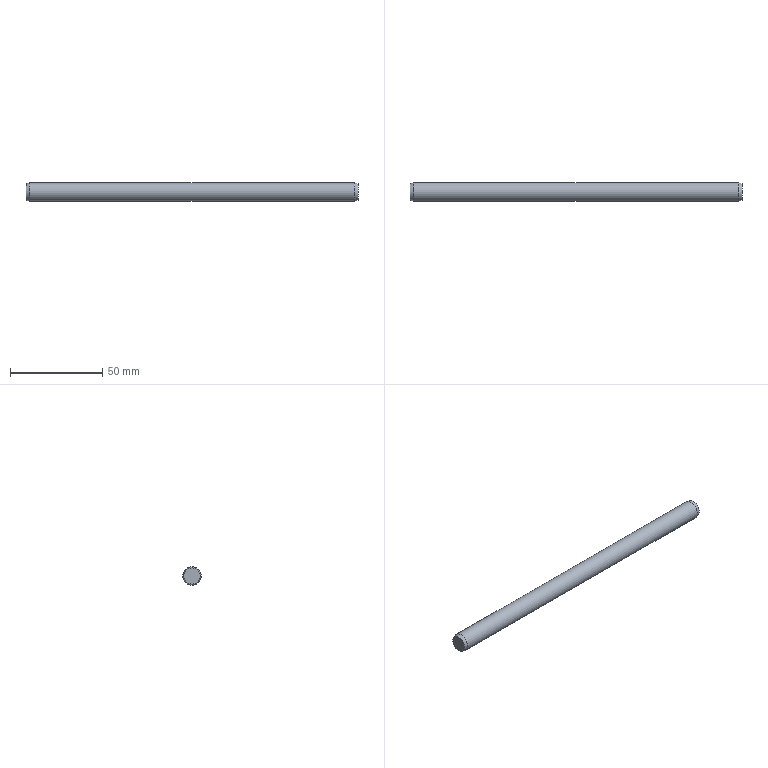Component | NX | HINGE | 1 solid | 5 faces | box 180 x 10 x 10 mm | volume 14105 mm3 | plane 2 | cone 2 | cylinder 1 | commonest cylinder face diameters 10 x1
STEP:
#1=CARTESIAN_POINT('',(0.,0.,0.));
#2=DIRECTION('',(0.,0.,1.));
#3=DIRECTION('',(1.,0.,0.));
#4=AXIS2_PLACEMENT_3D('',#1,#2,#3);
#5=CARTESIAN_POINT('',(-90.,140.,105.536));
#6=VERTEX_POINT('',#5);
#7=CARTESIAN_POINT('',(-90.,140.,110.));
#8=DIRECTION('',(-1.,0.,0.));
#9=DIRECTION('',(0.,0.,-1.));
#10=AXIS2_PLACEMENT_3D('',#7,#8,#9);
#11=CIRCLE('',#10,4.464);
#12=CARTESIAN_POINT('',(-90.,140.,110.));
#13=DIRECTION('',(-1.,0.,0.));
#14=DIRECTION('',(0.,0.,-1.));
#15=AXIS2_PLACEMENT_3D('',#12,#13,#14);
#16=PLANE('',#15);
#17=CARTESIAN_POINT('',(0.,0.));
#18=DIRECTION('',(1.,0.));
#19=AXIS2_PLACEMENT_2D('',#17,#18);
#20=CIRCLE('',#19,4.464);
#21=(GEOMETRIC_REPRESENTATION_CONTEXT(2)PARAMETRIC_REPRESENTATION_CONTEXT()REPRESENTATION_CONTEXT('',''));
#22=DEFINITIONAL_REPRESENTATION('',(#20),#21);
#23=PCURVE('',#16,#22);
#24=CARTESIAN_POINT('',(-90.,140.,110.));
#25=DIRECTION('',(1.,0.,0.));
#26=DIRECTION('',(0.,0.,1.));
#27=AXIS2_PLACEMENT_3D('',#24,#25,#26);
#28=CONICAL_SURFACE('',#27,4.464,0.2618);
#29=CARTESIAN_POINT('',(9.425,-0.));
#30=DIRECTION('',(-1.,0.));
#31=VECTOR('',#30,1.);
#32=LINE('',#29,#31);
#33=(GEOMETRIC_REPRESENTATION_CONTEXT(2)PARAMETRIC_REPRESENTATION_CONTEXT()REPRESENTATION_CONTEXT('',''));
#34=DEFINITIONAL_REPRESENTATION('',(#32),#33);
#35=PCURVE('',#28,#34);
#36=SURFACE_CURVE('',#11,(#23,#35),.PCURVE_S1.);
#37=EDGE_CURVE('',#6,#6,#36,.T.);
#38=ORIENTED_EDGE('',*,*,#37,.T.);
#39=EDGE_LOOP('',(#38));
#40=FACE_BOUND('',#39,.T.);
#41=ADVANCED_FACE('',(#40),#16,.T.);
#42=CARTESIAN_POINT('',(-88.,140.,105.));
#43=VERTEX_POINT('',#42);
#44=CARTESIAN_POINT('',(-88.,140.,110.));
#45=DIRECTION('',(-1.,0.,0.));
#46=DIRECTION('',(0.,0.,-1.));
#47=AXIS2_PLACEMENT_3D('',#44,#45,#46);
#48=CIRCLE('',#47,5.);
#49=CARTESIAN_POINT('',(9.425,2.));
#50=DIRECTION('',(-1.,0.));
#51=VECTOR('',#50,1.);
#52=LINE('',#49,#51);
#53=(GEOMETRIC_REPRESENTATION_CONTEXT(2)PARAMETRIC_REPRESENTATION_CONTEXT()REPRESENTATION_CONTEXT('',''));
#54=DEFINITIONAL_REPRESENTATION('',(#52),#53);
#55=PCURVE('',#28,#54);
#56=CARTESIAN_POINT('',(90.,140.,110.));
#57=DIRECTION('',(-1.,0.,0.));
#58=DIRECTION('',(0.,0.,-1.));
#59=AXIS2_PLACEMENT_3D('',#56,#57,#58);
#60=CYLINDRICAL_SURFACE('',#59,5.);
#61=CARTESIAN_POINT('',(0.,178.));
#62=DIRECTION('',(1.,0.));
#63=VECTOR('',#62,1.);
#64=LINE('',#61,#63);
#65=(GEOMETRIC_REPRESENTATION_CONTEXT(2)PARAMETRIC_REPRESENTATION_CONTEXT()REPRESENTATION_CONTEXT('',''));
#66=DEFINITIONAL_REPRESENTATION('',(#64),#65);
#67=PCURVE('',#60,#66);
#68=SURFACE_CURVE('',#48,(#55,#67),.PCURVE_S1.);
#69=EDGE_CURVE('',#43,#43,#68,.T.);
#70=ORIENTED_EDGE('',*,*,#69,.T.);
#71=CARTESIAN_POINT('',(-90.,140.,105.536));
#72=CARTESIAN_POINT('',(-88.,140.,105.));
#73=B_SPLINE_CURVE_WITH_KNOTS('',1,(#71,#72),.UNSPECIFIED.,.F.,.F.,(2,2),(-0.,2.071),.PIECEWISE_BEZIER_KNOTS.);
#74=CARTESIAN_POINT('',(3.142,0.));
#75=DIRECTION('',(0.,1.));
#76=VECTOR('',#75,1.);
#77=LINE('',#74,#76);
#78=(GEOMETRIC_REPRESENTATION_CONTEXT(2)PARAMETRIC_REPRESENTATION_CONTEXT()REPRESENTATION_CONTEXT('',''));
#79=DEFINITIONAL_REPRESENTATION('',(#77),#78);
#80=PCURVE('',#28,#79);
#81=CARTESIAN_POINT('',(9.425,0.));
#82=DIRECTION('',(0.,1.));
#83=VECTOR('',#82,1.);
#84=LINE('',#81,#83);
#85=(GEOMETRIC_REPRESENTATION_CONTEXT(2)PARAMETRIC_REPRESENTATION_CONTEXT()REPRESENTATION_CONTEXT('',''));
#86=DEFINITIONAL_REPRESENTATION('',(#84),#85);
#87=PCURVE('',#28,#86);
#88=SEAM_CURVE('',#73,(#80,#87),.PCURVE_S1.);
#89=EDGE_CURVE('',#6,#43,#88,.T.);
#90=ORIENTED_EDGE('',*,*,#89,.F.);
#91=ORIENTED_EDGE('',*,*,#37,.F.);
#92=ORIENTED_EDGE('',*,*,#89,.T.);
#93=EDGE_LOOP('',(#70,#90,#91,#92));
#94=FACE_BOUND('',#93,.T.);
#95=ADVANCED_FACE('',(#94),#28,.T.);
#96=CARTESIAN_POINT('',(88.,140.,105.));
#97=VERTEX_POINT('',#96);
#98=CARTESIAN_POINT('',(88.,140.,110.));
#99=DIRECTION('',(-1.,0.,0.));
#100=DIRECTION('',(0.,0.,-1.));
#101=AXIS2_PLACEMENT_3D('',#98,#99,#100);
#102=CIRCLE('',#101,5.);
#103=CARTESIAN_POINT('',(0.,2.));
#104=DIRECTION('',(1.,0.));
#105=VECTOR('',#104,1.);
#106=LINE('',#103,#105);
#107=(GEOMETRIC_REPRESENTATION_CONTEXT(2)PARAMETRIC_REPRESENTATION_CONTEXT()REPRESENTATION_CONTEXT('',''));
#108=DEFINITIONAL_REPRESENTATION('',(#106),#107);
#109=PCURVE('',#60,#108);
#110=CARTESIAN_POINT('',(88.,140.,110.));
#111=DIRECTION('',(-1.,0.,0.));
#112=DIRECTION('',(0.,0.,-1.));
#113=AXIS2_PLACEMENT_3D('',#110,#111,#112);
#114=CONICAL_SURFACE('',#113,5.,0.2618);
#115=CARTESIAN_POINT('',(0.,-0.));
#116=DIRECTION('',(1.,0.));
#117=VECTOR('',#116,1.);
#118=LINE('',#115,#117);
#119=(GEOMETRIC_REPRESENTATION_CONTEXT(2)PARAMETRIC_REPRESENTATION_CONTEXT()REPRESENTATION_CONTEXT('',''));
#120=DEFINITIONAL_REPRESENTATION('',(#118),#119);
#121=PCURVE('',#114,#120);
#122=SURFACE_CURVE('',#102,(#109,#121),.PCURVE_S1.);
#123=EDGE_CURVE('',#97,#97,#122,.T.);
#124=ORIENTED_EDGE('',*,*,#123,.T.);
#125=CARTESIAN_POINT('',(88.,140.,105.));
#126=CARTESIAN_POINT('',(-88.,140.,105.));
#127=B_SPLINE_CURVE_WITH_KNOTS('',1,(#125,#126),.UNSPECIFIED.,.F.,.F.,(2,2),(2.,178.),.PIECEWISE_BEZIER_KNOTS.);
#128=CARTESIAN_POINT('',(6.283,0.));
#129=DIRECTION('',(0.,1.));
#130=VECTOR('',#129,1.);
#131=LINE('',#128,#130);
#132=(GEOMETRIC_REPRESENTATION_CONTEXT(2)PARAMETRIC_REPRESENTATION_CONTEXT()REPRESENTATION_CONTEXT('',''));
#133=DEFINITIONAL_REPRESENTATION('',(#131),#132);
#134=PCURVE('',#60,#133);
#135=CARTESIAN_POINT('',(0.,0.));
#136=DIRECTION('',(0.,1.));
#137=VECTOR('',#136,1.);
#138=LINE('',#135,#137);
#139=(GEOMETRIC_REPRESENTATION_CONTEXT(2)PARAMETRIC_REPRESENTATION_CONTEXT()REPRESENTATION_CONTEXT('',''));
#140=DEFINITIONAL_REPRESENTATION('',(#138),#139);
#141=PCURVE('',#60,#140);
#142=SEAM_CURVE('',#127,(#134,#141),.PCURVE_S1.);
#143=EDGE_CURVE('',#97,#43,#142,.T.);
#144=ORIENTED_EDGE('',*,*,#143,.T.);
#145=ORIENTED_EDGE('',*,*,#69,.F.);
#146=ORIENTED_EDGE('',*,*,#143,.F.);
#147=EDGE_LOOP('',(#124,#144,#145,#146));
#148=FACE_BOUND('',#147,.T.);
#149=ADVANCED_FACE('',(#148),#60,.T.);
#150=CARTESIAN_POINT('',(90.,140.,105.536));
#151=VERTEX_POINT('',#150);
#152=CARTESIAN_POINT('',(90.,140.,110.));
#153=DIRECTION('',(-1.,0.,0.));
#154=DIRECTION('',(0.,0.,-1.));
#155=AXIS2_PLACEMENT_3D('',#152,#153,#154);
#156=CIRCLE('',#155,4.464);
#157=CARTESIAN_POINT('',(0.,-2.));
#158=DIRECTION('',(1.,0.));
#159=VECTOR('',#158,1.);
#160=LINE('',#157,#159);
#161=(GEOMETRIC_REPRESENTATION_CONTEXT(2)PARAMETRIC_REPRESENTATION_CONTEXT()REPRESENTATION_CONTEXT('',''));
#162=DEFINITIONAL_REPRESENTATION('',(#160),#161);
#163=PCURVE('',#114,#162);
#164=CARTESIAN_POINT('',(90.,140.,114.464));
#165=DIRECTION('',(1.,0.,0.));
#166=DIRECTION('',(0.,0.,1.));
#167=AXIS2_PLACEMENT_3D('',#164,#165,#166);
#168=PLANE('',#167);
#169=CARTESIAN_POINT('',(-8.928,0.));
#170=CARTESIAN_POINT('',(-8.928,7.732));
#171=CARTESIAN_POINT('',(-2.232,3.866));
#172=CARTESIAN_POINT('',(4.464,0.));
#173=CARTESIAN_POINT('',(-2.232,-3.866));
#174=CARTESIAN_POINT('',(-8.928,-7.732));
#175=CARTESIAN_POINT('',(-8.928,0.));
#176=(BOUNDED_CURVE()B_SPLINE_CURVE(2,(#169,#170,#171,#172,#173,#174,#175),.UNSPECIFIED.,.T.,.F.)B_SPLINE_CURVE_WITH_KNOTS((1,2,2,2,2,1),(-2.094,0.,2.094,4.189,6.283,8.378),.UNSPECIFIED.)CURVE()GEOMETRIC_REPRESENTATION_ITEM()RATIONAL_B_SPLINE_CURVE((1.,0.5,1.,0.5,1.,0.5,1.))REPRESENTATION_ITEM(''));
#177=(GEOMETRIC_REPRESENTATION_CONTEXT(2)PARAMETRIC_REPRESENTATION_CONTEXT()REPRESENTATION_CONTEXT('',''));
#178=DEFINITIONAL_REPRESENTATION('',(#176),#177);
#179=PCURVE('',#168,#178);
#180=SURFACE_CURVE('',#156,(#163,#179),.PCURVE_S1.);
#181=EDGE_CURVE('',#151,#151,#180,.T.);
#182=ORIENTED_EDGE('',*,*,#181,.T.);
#183=CARTESIAN_POINT('',(90.,140.,105.536));
#184=CARTESIAN_POINT('',(88.,140.,105.));
#185=B_SPLINE_CURVE_WITH_KNOTS('',1,(#183,#184),.UNSPECIFIED.,.F.,.F.,(2,2),(-2.071,-0.),.PIECEWISE_BEZIER_KNOTS.);
#186=CARTESIAN_POINT('',(6.283,0.));
#187=DIRECTION('',(0.,1.));
#188=VECTOR('',#187,1.);
#189=LINE('',#186,#188);
#190=(GEOMETRIC_REPRESENTATION_CONTEXT(2)PARAMETRIC_REPRESENTATION_CONTEXT()REPRESENTATION_CONTEXT('',''));
#191=DEFINITIONAL_REPRESENTATION('',(#189),#190);
#192=PCURVE('',#114,#191);
#193=CARTESIAN_POINT('',(0.,0.));
#194=DIRECTION('',(0.,1.));
#195=VECTOR('',#194,1.);
#196=LINE('',#193,#195);
#197=(GEOMETRIC_REPRESENTATION_CONTEXT(2)PARAMETRIC_REPRESENTATION_CONTEXT()REPRESENTATION_CONTEXT('',''));
#198=DEFINITIONAL_REPRESENTATION('',(#196),#197);
#199=PCURVE('',#114,#198);
#200=SEAM_CURVE('',#185,(#192,#199),.PCURVE_S1.);
#201=EDGE_CURVE('',#151,#97,#200,.T.);
#202=ORIENTED_EDGE('',*,*,#201,.T.);
#203=ORIENTED_EDGE('',*,*,#123,.F.);
#204=ORIENTED_EDGE('',*,*,#201,.F.);
#205=EDGE_LOOP('',(#182,#202,#203,#204));
#206=FACE_BOUND('',#205,.T.);
#207=ADVANCED_FACE('',(#206),#114,.T.);
#208=ORIENTED_EDGE('',*,*,#181,.F.);
#209=EDGE_LOOP('',(#208));
#210=FACE_BOUND('',#209,.T.);
#211=ADVANCED_FACE('',(#210),#168,.T.);
#212=CLOSED_SHELL('',(#41,#95,#149,#207,#211));
#213=MANIFOLD_SOLID_BREP('',#212);
#214=(LENGTH_UNIT()NAMED_UNIT(*)SI_UNIT(.MILLI.,.METRE.));
#215=UNCERTAINTY_MEASURE_WITH_UNIT(LENGTH_MEASURE(0.00001),#214,'','');
#216=(NAMED_UNIT(*)PLANE_ANGLE_UNIT()SI_UNIT($,.RADIAN.));
#217=(NAMED_UNIT(*)SI_UNIT($,.STERADIAN.)SOLID_ANGLE_UNIT());
#218=(GEOMETRIC_REPRESENTATION_CONTEXT(3)GLOBAL_UNCERTAINTY_ASSIGNED_CONTEXT((#215))GLOBAL_UNIT_ASSIGNED_CONTEXT((#214,#216,#217))REPRESENTATION_CONTEXT('',''));
#219=ADVANCED_BREP_SHAPE_REPRESENTATION('',(#4,#213),#218);